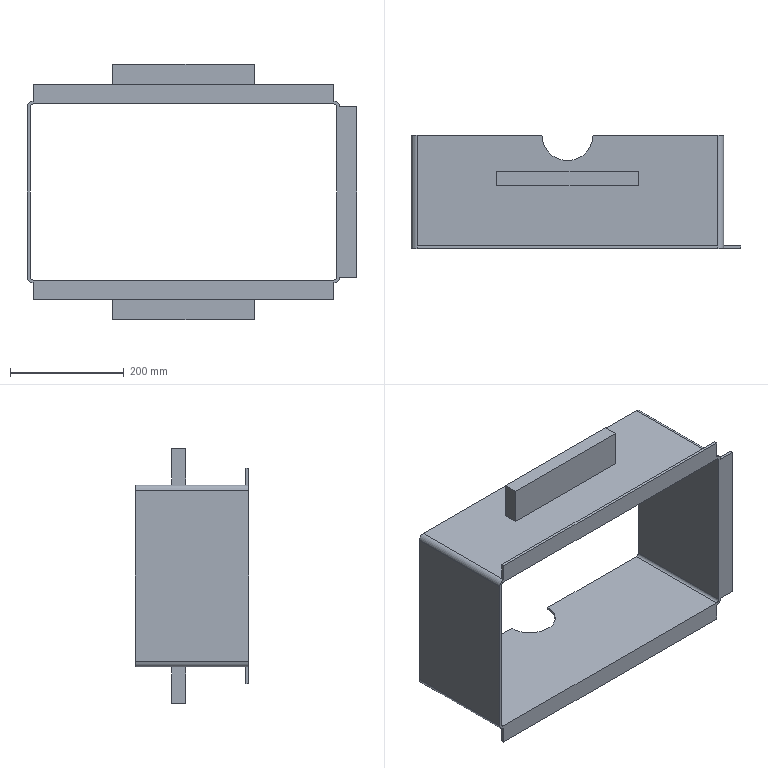Component | SolidWorks | MiddleHousing-1_MiddleHousing1-1 | 1 solid | 43 faces | volume 2691815 mm3 | plane 33 | cylinder 10 | commonest cylinder face diameters 10 x4 20 x4 90 x2